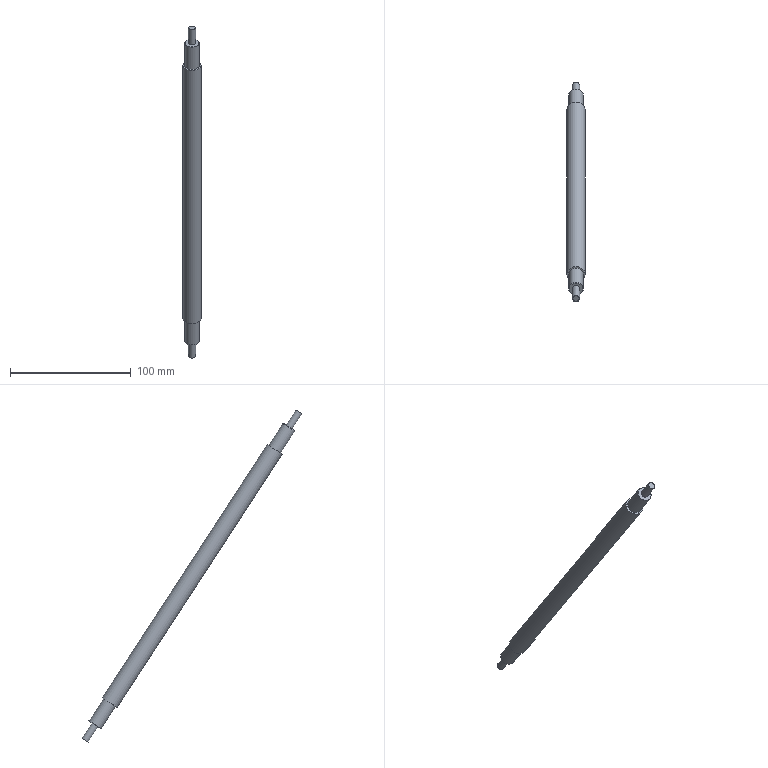Component | NX | BOTTOM_ROD | 1 solid | 13 faces | box 15 x 181.81 x 274.63 mm | volume 50002 mm3 | plane 6 | cylinder 5 | cone 2 | commonest cylinder face diameters 12 x2 6 x2 15 x1
STEP:
#1=CARTESIAN_POINT('',(0.,0.,0.));
#2=DIRECTION('',(0.,0.,1.));
#3=DIRECTION('',(1.,0.,0.));
#4=AXIS2_PLACEMENT_3D('',#1,#2,#3);
#5=CARTESIAN_POINT('',(319.193,-152.841,329.605));
#6=VERTEX_POINT('',#5);
#7=CARTESIAN_POINT('',(311.693,-152.841,329.605));
#8=DIRECTION('',(0.,-0.5459,0.8379));
#9=DIRECTION('',(1.,0.,0.));
#10=AXIS2_PLACEMENT_3D('',#7,#8,#9);
#11=CIRCLE('',#10,7.5);
#12=CARTESIAN_POINT('',(311.693,-152.841,329.605));
#13=DIRECTION('',(0.,0.5459,-0.8379));
#14=DIRECTION('',(-1.,0.,0.));
#15=AXIS2_PLACEMENT_3D('',#12,#13,#14);
#16=CYLINDRICAL_SURFACE('',#15,7.5);
#17=CARTESIAN_POINT('',(9.425,0.));
#18=DIRECTION('',(-1.,0.));
#19=VECTOR('',#18,1.);
#20=LINE('',#17,#19);
#21=(GEOMETRIC_REPRESENTATION_CONTEXT(2)PARAMETRIC_REPRESENTATION_CONTEXT()REPRESENTATION_CONTEXT('',''));
#22=DEFINITIONAL_REPRESENTATION('',(#20),#21);
#23=PCURVE('',#16,#22);
#24=CARTESIAN_POINT('',(311.693,-152.841,329.605));
#25=DIRECTION('',(0.,-0.5459,0.8379));
#26=DIRECTION('',(1.,0.,0.));
#27=AXIS2_PLACEMENT_3D('',#24,#25,#26);
#28=PLANE('',#27);
#29=CARTESIAN_POINT('',(0.,0.));
#30=DIRECTION('',(1.,0.));
#31=AXIS2_PLACEMENT_2D('',#29,#30);
#32=CIRCLE('',#31,7.5);
#33=(GEOMETRIC_REPRESENTATION_CONTEXT(2)PARAMETRIC_REPRESENTATION_CONTEXT()REPRESENTATION_CONTEXT('',''));
#34=DEFINITIONAL_REPRESENTATION('',(#32),#33);
#35=PCURVE('',#28,#34);
#36=SURFACE_CURVE('',#11,(#23,#35),.PCURVE_S1.);
#37=EDGE_CURVE('',#6,#6,#36,.T.);
#38=ORIENTED_EDGE('',*,*,#37,.F.);
#39=CARTESIAN_POINT('',(319.193,-16.376,120.136));
#40=VERTEX_POINT('',#39);
#41=CARTESIAN_POINT('',(319.193,-152.841,329.605));
#42=CARTESIAN_POINT('',(319.193,-16.376,120.136));
#43=B_SPLINE_CURVE_WITH_KNOTS('',1,(#41,#42),.UNSPECIFIED.,.F.,.F.,(2,2),(0.,250.),.PIECEWISE_BEZIER_KNOTS.);
#44=CARTESIAN_POINT('',(9.425,0.));
#45=DIRECTION('',(0.,1.));
#46=VECTOR('',#45,1.);
#47=LINE('',#44,#46);
#48=(GEOMETRIC_REPRESENTATION_CONTEXT(2)PARAMETRIC_REPRESENTATION_CONTEXT()REPRESENTATION_CONTEXT('',''));
#49=DEFINITIONAL_REPRESENTATION('',(#47),#48);
#50=PCURVE('',#16,#49);
#51=CARTESIAN_POINT('',(3.142,0.));
#52=DIRECTION('',(0.,1.));
#53=VECTOR('',#52,1.);
#54=LINE('',#51,#53);
#55=(GEOMETRIC_REPRESENTATION_CONTEXT(2)PARAMETRIC_REPRESENTATION_CONTEXT()REPRESENTATION_CONTEXT('',''));
#56=DEFINITIONAL_REPRESENTATION('',(#54),#55);
#57=PCURVE('',#16,#56);
#58=SEAM_CURVE('',#43,(#50,#57),.PCURVE_S1.);
#59=EDGE_CURVE('',#6,#40,#58,.T.);
#60=ORIENTED_EDGE('',*,*,#59,.T.);
#61=CARTESIAN_POINT('',(311.693,-16.376,120.136));
#62=DIRECTION('',(0.,-0.5459,0.8379));
#63=DIRECTION('',(1.,0.,0.));
#64=AXIS2_PLACEMENT_3D('',#61,#62,#63);
#65=CIRCLE('',#64,7.5);
#66=CARTESIAN_POINT('',(9.425,250.));
#67=DIRECTION('',(-1.,0.));
#68=VECTOR('',#67,1.);
#69=LINE('',#66,#68);
#70=(GEOMETRIC_REPRESENTATION_CONTEXT(2)PARAMETRIC_REPRESENTATION_CONTEXT()REPRESENTATION_CONTEXT('',''));
#71=DEFINITIONAL_REPRESENTATION('',(#69),#70);
#72=PCURVE('',#16,#71);
#73=CARTESIAN_POINT('',(311.693,-16.376,120.136));
#74=DIRECTION('',(0.,-0.5459,0.8379));
#75=DIRECTION('',(1.,0.,0.));
#76=AXIS2_PLACEMENT_3D('',#73,#74,#75);
#77=PLANE('',#76);
#78=CARTESIAN_POINT('',(0.,0.));
#79=DIRECTION('',(1.,0.));
#80=AXIS2_PLACEMENT_2D('',#78,#79);
#81=CIRCLE('',#80,7.5);
#82=(GEOMETRIC_REPRESENTATION_CONTEXT(2)PARAMETRIC_REPRESENTATION_CONTEXT()REPRESENTATION_CONTEXT('',''));
#83=DEFINITIONAL_REPRESENTATION('',(#81),#82);
#84=PCURVE('',#77,#83);
#85=SURFACE_CURVE('',#65,(#72,#84),.PCURVE_S1.);
#86=EDGE_CURVE('',#40,#40,#85,.T.);
#87=ORIENTED_EDGE('',*,*,#86,.T.);
#88=ORIENTED_EDGE('',*,*,#59,.F.);
#89=EDGE_LOOP('',(#38,#60,#87,#88));
#90=FACE_BOUND('',#89,.T.);
#91=ADVANCED_FACE('',(#90),#16,.T.);
#92=CARTESIAN_POINT('',(317.693,-152.841,329.605));
#93=VERTEX_POINT('',#92);
#94=CARTESIAN_POINT('',(311.693,-152.841,329.605));
#95=DIRECTION('',(0.,-0.5459,0.8379));
#96=DIRECTION('',(1.,0.,0.));
#97=AXIS2_PLACEMENT_3D('',#94,#95,#96);
#98=CIRCLE('',#97,6.);
#99=CARTESIAN_POINT('',(0.,0.));
#100=DIRECTION('',(1.,0.));
#101=AXIS2_PLACEMENT_2D('',#99,#100);
#102=CIRCLE('',#101,6.);
#103=(GEOMETRIC_REPRESENTATION_CONTEXT(2)PARAMETRIC_REPRESENTATION_CONTEXT()REPRESENTATION_CONTEXT('',''));
#104=DEFINITIONAL_REPRESENTATION('',(#102),#103);
#105=PCURVE('',#28,#104);
#106=CARTESIAN_POINT('',(311.693,-164.85,348.038));
#107=DIRECTION('',(0.,0.5459,-0.8379));
#108=DIRECTION('',(-1.,0.,0.));
#109=AXIS2_PLACEMENT_3D('',#106,#107,#108);
#110=CYLINDRICAL_SURFACE('',#109,6.);
#111=CARTESIAN_POINT('',(9.425,22.));
#112=DIRECTION('',(-1.,0.));
#113=VECTOR('',#112,1.);
#114=LINE('',#111,#113);
#115=(GEOMETRIC_REPRESENTATION_CONTEXT(2)PARAMETRIC_REPRESENTATION_CONTEXT()REPRESENTATION_CONTEXT('',''));
#116=DEFINITIONAL_REPRESENTATION('',(#114),#115);
#117=PCURVE('',#110,#116);
#118=SURFACE_CURVE('',#98,(#105,#117),.PCURVE_S1.);
#119=EDGE_CURVE('',#93,#93,#118,.T.);
#120=ORIENTED_EDGE('',*,*,#119,.F.);
#121=EDGE_LOOP('',(#120));
#122=FACE_BOUND('',#121,.T.);
#123=ORIENTED_EDGE('',*,*,#37,.T.);
#124=EDGE_LOOP('',(#123));
#125=FACE_BOUND('',#124,.T.);
#126=ADVANCED_FACE('',(#122,#125),#28,.T.);
#127=CARTESIAN_POINT('',(317.693,-16.376,120.136));
#128=VERTEX_POINT('',#127);
#129=CARTESIAN_POINT('',(311.693,-16.376,120.136));
#130=DIRECTION('',(0.,-0.5459,0.8379));
#131=DIRECTION('',(1.,0.,0.));
#132=AXIS2_PLACEMENT_3D('',#129,#130,#131);
#133=CIRCLE('',#132,6.);
#134=CARTESIAN_POINT('',(0.,0.));
#135=DIRECTION('',(1.,0.));
#136=AXIS2_PLACEMENT_2D('',#134,#135);
#137=CIRCLE('',#136,6.);
#138=(GEOMETRIC_REPRESENTATION_CONTEXT(2)PARAMETRIC_REPRESENTATION_CONTEXT()REPRESENTATION_CONTEXT('',''));
#139=DEFINITIONAL_REPRESENTATION('',(#137),#138);
#140=PCURVE('',#77,#139);
#141=CARTESIAN_POINT('',(311.693,-4.367,101.703));
#142=DIRECTION('',(0.,-0.5459,0.8379));
#143=DIRECTION('',(1.,0.,0.));
#144=AXIS2_PLACEMENT_3D('',#141,#142,#143);
#145=CYLINDRICAL_SURFACE('',#144,6.);
#146=CARTESIAN_POINT('',(0.,22.));
#147=DIRECTION('',(1.,0.));
#148=VECTOR('',#147,1.);
#149=LINE('',#146,#148);
#150=(GEOMETRIC_REPRESENTATION_CONTEXT(2)PARAMETRIC_REPRESENTATION_CONTEXT()REPRESENTATION_CONTEXT('',''));
#151=DEFINITIONAL_REPRESENTATION('',(#149),#150);
#152=PCURVE('',#145,#151);
#153=SURFACE_CURVE('',#133,(#140,#152),.PCURVE_S1.);
#154=EDGE_CURVE('',#128,#128,#153,.T.);
#155=ORIENTED_EDGE('',*,*,#154,.T.);
#156=EDGE_LOOP('',(#155));
#157=FACE_BOUND('',#156,.T.);
#158=ORIENTED_EDGE('',*,*,#86,.F.);
#159=EDGE_LOOP('',(#158));
#160=FACE_BOUND('',#159,.T.);
#161=ADVANCED_FACE('',(#157,#160),#77,.F.);
#162=CARTESIAN_POINT('',(317.693,-164.714,347.829));
#163=VERTEX_POINT('',#162);
#164=CARTESIAN_POINT('',(311.693,-164.714,347.829));
#165=DIRECTION('',(0.,0.5459,-0.8379));
#166=DIRECTION('',(1.,0.,0.));
#167=AXIS2_PLACEMENT_3D('',#164,#165,#166);
#168=CIRCLE('',#167,6.);
#169=CARTESIAN_POINT('',(3.142,0.25));
#170=DIRECTION('',(1.,0.));
#171=VECTOR('',#170,1.);
#172=LINE('',#169,#171);
#173=(GEOMETRIC_REPRESENTATION_CONTEXT(2)PARAMETRIC_REPRESENTATION_CONTEXT()REPRESENTATION_CONTEXT('',''));
#174=DEFINITIONAL_REPRESENTATION('',(#172),#173);
#175=PCURVE('',#110,#174);
#176=CARTESIAN_POINT('',(311.693,-164.85,348.038));
#177=DIRECTION('',(0.,0.5459,-0.8379));
#178=DIRECTION('',(-1.,0.,0.));
#179=AXIS2_PLACEMENT_3D('',#176,#177,#178);
#180=CONICAL_SURFACE('',#179,5.75,0.7854);
#181=CARTESIAN_POINT('',(3.142,0.25));
#182=DIRECTION('',(1.,0.));
#183=VECTOR('',#182,1.);
#184=LINE('',#181,#183);
#185=(GEOMETRIC_REPRESENTATION_CONTEXT(2)PARAMETRIC_REPRESENTATION_CONTEXT()REPRESENTATION_CONTEXT('',''));
#186=DEFINITIONAL_REPRESENTATION('',(#184),#185);
#187=PCURVE('',#180,#186);
#188=SURFACE_CURVE('',#168,(#175,#187),.PCURVE_S1.);
#189=EDGE_CURVE('',#163,#163,#188,.T.);
#190=ORIENTED_EDGE('',*,*,#189,.T.);
#191=CARTESIAN_POINT('',(317.693,-164.714,347.829));
#192=CARTESIAN_POINT('',(317.693,-152.841,329.605));
#193=B_SPLINE_CURVE_WITH_KNOTS('',1,(#191,#192),.UNSPECIFIED.,.F.,.F.,(2,2),(0.25,22.),.PIECEWISE_BEZIER_KNOTS.);
#194=CARTESIAN_POINT('',(9.425,0.));
#195=DIRECTION('',(0.,1.));
#196=VECTOR('',#195,1.);
#197=LINE('',#194,#196);
#198=(GEOMETRIC_REPRESENTATION_CONTEXT(2)PARAMETRIC_REPRESENTATION_CONTEXT()REPRESENTATION_CONTEXT('',''));
#199=DEFINITIONAL_REPRESENTATION('',(#197),#198);
#200=PCURVE('',#110,#199);
#201=CARTESIAN_POINT('',(3.142,0.));
#202=DIRECTION('',(0.,1.));
#203=VECTOR('',#202,1.);
#204=LINE('',#201,#203);
#205=(GEOMETRIC_REPRESENTATION_CONTEXT(2)PARAMETRIC_REPRESENTATION_CONTEXT()REPRESENTATION_CONTEXT('',''));
#206=DEFINITIONAL_REPRESENTATION('',(#204),#205);
#207=PCURVE('',#110,#206);
#208=SEAM_CURVE('',#193,(#200,#207),.PCURVE_S1.);
#209=EDGE_CURVE('',#163,#93,#208,.T.);
#210=ORIENTED_EDGE('',*,*,#209,.T.);
#211=ORIENTED_EDGE('',*,*,#119,.T.);
#212=ORIENTED_EDGE('',*,*,#209,.F.);
#213=EDGE_LOOP('',(#190,#210,#211,#212));
#214=FACE_BOUND('',#213,.T.);
#215=ADVANCED_FACE('',(#214),#110,.T.);
#216=CARTESIAN_POINT('',(317.443,-164.85,348.038));
#217=VERTEX_POINT('',#216);
#218=CARTESIAN_POINT('',(311.693,-164.85,348.038));
#219=DIRECTION('',(0.,-0.5459,0.8379));
#220=DIRECTION('',(1.,0.,0.));
#221=AXIS2_PLACEMENT_3D('',#218,#219,#220);
#222=CIRCLE('',#221,5.75);
#223=CARTESIAN_POINT('',(311.693,-164.85,348.038));
#224=DIRECTION('',(0.,-0.5459,0.8379));
#225=DIRECTION('',(1.,0.,0.));
#226=AXIS2_PLACEMENT_3D('',#223,#224,#225);
#227=PLANE('',#226);
#228=CARTESIAN_POINT('',(0.,0.));
#229=DIRECTION('',(1.,0.));
#230=AXIS2_PLACEMENT_2D('',#228,#229);
#231=CIRCLE('',#230,5.75);
#232=(GEOMETRIC_REPRESENTATION_CONTEXT(2)PARAMETRIC_REPRESENTATION_CONTEXT()REPRESENTATION_CONTEXT('',''));
#233=DEFINITIONAL_REPRESENTATION('',(#231),#232);
#234=PCURVE('',#227,#233);
#235=CARTESIAN_POINT('',(9.425,0.));
#236=DIRECTION('',(-1.,0.));
#237=VECTOR('',#236,1.);
#238=LINE('',#235,#237);
#239=(GEOMETRIC_REPRESENTATION_CONTEXT(2)PARAMETRIC_REPRESENTATION_CONTEXT()REPRESENTATION_CONTEXT('',''));
#240=DEFINITIONAL_REPRESENTATION('',(#238),#239);
#241=PCURVE('',#180,#240);
#242=SURFACE_CURVE('',#222,(#234,#241),.PCURVE_S1.);
#243=EDGE_CURVE('',#217,#217,#242,.T.);
#244=ORIENTED_EDGE('',*,*,#243,.T.);
#245=EDGE_LOOP('',(#244));
#246=FACE_BOUND('',#245,.T.);
#247=CARTESIAN_POINT('',(314.693,-164.85,348.038));
#248=VERTEX_POINT('',#247);
#249=CARTESIAN_POINT('',(311.693,-164.85,348.038));
#250=DIRECTION('',(0.,-0.5459,0.8379));
#251=DIRECTION('',(1.,0.,0.));
#252=AXIS2_PLACEMENT_3D('',#249,#250,#251);
#253=CIRCLE('',#252,3.);
#254=CARTESIAN_POINT('',(0.,0.));
#255=DIRECTION('',(1.,0.));
#256=AXIS2_PLACEMENT_2D('',#254,#255);
#257=CIRCLE('',#256,3.);
#258=(GEOMETRIC_REPRESENTATION_CONTEXT(2)PARAMETRIC_REPRESENTATION_CONTEXT()REPRESENTATION_CONTEXT('',''));
#259=DEFINITIONAL_REPRESENTATION('',(#257),#258);
#260=PCURVE('',#227,#259);
#261=CARTESIAN_POINT('',(311.693,-173.038,360.607));
#262=DIRECTION('',(0.,0.5459,-0.8379));
#263=DIRECTION('',(-1.,0.,0.));
#264=AXIS2_PLACEMENT_3D('',#261,#262,#263);
#265=CYLINDRICAL_SURFACE('',#264,3.);
#266=CARTESIAN_POINT('',(9.425,15.));
#267=DIRECTION('',(-1.,0.));
#268=VECTOR('',#267,1.);
#269=LINE('',#266,#268);
#270=(GEOMETRIC_REPRESENTATION_CONTEXT(2)PARAMETRIC_REPRESENTATION_CONTEXT()REPRESENTATION_CONTEXT('',''));
#271=DEFINITIONAL_REPRESENTATION('',(#269),#270);
#272=PCURVE('',#265,#271);
#273=SURFACE_CURVE('',#253,(#260,#272),.PCURVE_S1.);
#274=EDGE_CURVE('',#248,#248,#273,.T.);
#275=ORIENTED_EDGE('',*,*,#274,.F.);
#276=EDGE_LOOP('',(#275));
#277=FACE_BOUND('',#276,.T.);
#278=ADVANCED_FACE('',(#246,#277),#227,.T.);
#279=CARTESIAN_POINT('',(314.693,-172.959,360.486));
#280=VERTEX_POINT('',#279);
#281=CARTESIAN_POINT('',(311.693,-172.959,360.486));
#282=DIRECTION('',(0.,0.5459,-0.8379));
#283=DIRECTION('',(1.,0.,0.));
#284=AXIS2_PLACEMENT_3D('',#281,#282,#283);
#285=CIRCLE('',#284,3.);
#286=CARTESIAN_POINT('',(3.142,0.1443));
#287=DIRECTION('',(1.,0.));
#288=VECTOR('',#287,1.);
#289=LINE('',#286,#288);
#290=(GEOMETRIC_REPRESENTATION_CONTEXT(2)PARAMETRIC_REPRESENTATION_CONTEXT()REPRESENTATION_CONTEXT('',''));
#291=DEFINITIONAL_REPRESENTATION('',(#289),#290);
#292=PCURVE('',#265,#291);
#293=CARTESIAN_POINT('',(311.693,-173.038,360.607));
#294=DIRECTION('',(0.,0.5459,-0.8379));
#295=DIRECTION('',(-1.,0.,0.));
#296=AXIS2_PLACEMENT_3D('',#293,#294,#295);
#297=CONICAL_SURFACE('',#296,2.75,1.047);
#298=CARTESIAN_POINT('',(3.142,0.1443));
#299=DIRECTION('',(1.,0.));
#300=VECTOR('',#299,1.);
#301=LINE('',#298,#300);
#302=(GEOMETRIC_REPRESENTATION_CONTEXT(2)PARAMETRIC_REPRESENTATION_CONTEXT()REPRESENTATION_CONTEXT('',''));
#303=DEFINITIONAL_REPRESENTATION('',(#301),#302);
#304=PCURVE('',#297,#303);
#305=SURFACE_CURVE('',#285,(#292,#304),.PCURVE_S1.);
#306=EDGE_CURVE('',#280,#280,#305,.T.);
#307=ORIENTED_EDGE('',*,*,#306,.T.);
#308=CARTESIAN_POINT('',(314.693,-172.959,360.486));
#309=CARTESIAN_POINT('',(314.693,-164.85,348.038));
#310=B_SPLINE_CURVE_WITH_KNOTS('',1,(#308,#309),.UNSPECIFIED.,.F.,.F.,(2,2),(0.1443,15.),.PIECEWISE_BEZIER_KNOTS.);
#311=CARTESIAN_POINT('',(9.425,0.));
#312=DIRECTION('',(0.,1.));
#313=VECTOR('',#312,1.);
#314=LINE('',#311,#313);
#315=(GEOMETRIC_REPRESENTATION_CONTEXT(2)PARAMETRIC_REPRESENTATION_CONTEXT()REPRESENTATION_CONTEXT('',''));
#316=DEFINITIONAL_REPRESENTATION('',(#314),#315);
#317=PCURVE('',#265,#316);
#318=CARTESIAN_POINT('',(3.142,0.));
#319=DIRECTION('',(0.,1.));
#320=VECTOR('',#319,1.);
#321=LINE('',#318,#320);
#322=(GEOMETRIC_REPRESENTATION_CONTEXT(2)PARAMETRIC_REPRESENTATION_CONTEXT()REPRESENTATION_CONTEXT('',''));
#323=DEFINITIONAL_REPRESENTATION('',(#321),#322);
#324=PCURVE('',#265,#323);
#325=SEAM_CURVE('',#310,(#317,#324),.PCURVE_S1.);
#326=EDGE_CURVE('',#280,#248,#325,.T.);
#327=ORIENTED_EDGE('',*,*,#326,.T.);
#328=ORIENTED_EDGE('',*,*,#274,.T.);
#329=ORIENTED_EDGE('',*,*,#326,.F.);
#330=EDGE_LOOP('',(#307,#327,#328,#329));
#331=FACE_BOUND('',#330,.T.);
#332=ADVANCED_FACE('',(#331),#265,.T.);
#333=CARTESIAN_POINT('',(314.443,-173.038,360.607));
#334=VERTEX_POINT('',#333);
#335=CARTESIAN_POINT('',(311.693,-173.038,360.607));
#336=DIRECTION('',(0.,-0.5459,0.8379));
#337=DIRECTION('',(1.,0.,0.));
#338=AXIS2_PLACEMENT_3D('',#335,#336,#337);
#339=CIRCLE('',#338,2.75);
#340=CARTESIAN_POINT('',(311.693,-173.038,360.607));
#341=DIRECTION('',(0.,-0.5459,0.8379));
#342=DIRECTION('',(1.,0.,0.));
#343=AXIS2_PLACEMENT_3D('',#340,#341,#342);
#344=PLANE('',#343);
#345=CARTESIAN_POINT('',(0.,0.));
#346=DIRECTION('',(1.,0.));
#347=AXIS2_PLACEMENT_2D('',#345,#346);
#348=CIRCLE('',#347,2.75);
#349=(GEOMETRIC_REPRESENTATION_CONTEXT(2)PARAMETRIC_REPRESENTATION_CONTEXT()REPRESENTATION_CONTEXT('',''));
#350=DEFINITIONAL_REPRESENTATION('',(#348),#349);
#351=PCURVE('',#344,#350);
#352=CARTESIAN_POINT('',(9.425,0.));
#353=DIRECTION('',(-1.,0.));
#354=VECTOR('',#353,1.);
#355=LINE('',#352,#354);
#356=(GEOMETRIC_REPRESENTATION_CONTEXT(2)PARAMETRIC_REPRESENTATION_CONTEXT()REPRESENTATION_CONTEXT('',''));
#357=DEFINITIONAL_REPRESENTATION('',(#355),#356);
#358=PCURVE('',#297,#357);
#359=SURFACE_CURVE('',#339,(#351,#358),.PCURVE_S1.);
#360=EDGE_CURVE('',#334,#334,#359,.T.);
#361=ORIENTED_EDGE('',*,*,#360,.T.);
#362=EDGE_LOOP('',(#361));
#363=FACE_BOUND('',#362,.T.);
#364=ADVANCED_FACE('',(#363),#344,.T.);
#365=ORIENTED_EDGE('',*,*,#306,.F.);
#366=CARTESIAN_POINT('',(314.443,-173.038,360.607));
#367=CARTESIAN_POINT('',(314.693,-172.959,360.486));
#368=B_SPLINE_CURVE_WITH_KNOTS('',1,(#366,#367),.UNSPECIFIED.,.F.,.F.,(2,2),(0.,0.2887),.PIECEWISE_BEZIER_KNOTS.);
#369=CARTESIAN_POINT('',(3.142,0.));
#370=DIRECTION('',(0.,1.));
#371=VECTOR('',#370,1.);
#372=LINE('',#369,#371);
#373=(GEOMETRIC_REPRESENTATION_CONTEXT(2)PARAMETRIC_REPRESENTATION_CONTEXT()REPRESENTATION_CONTEXT('',''));
#374=DEFINITIONAL_REPRESENTATION('',(#372),#373);
#375=PCURVE('',#297,#374);
#376=CARTESIAN_POINT('',(9.425,0.));
#377=DIRECTION('',(0.,1.));
#378=VECTOR('',#377,1.);
#379=LINE('',#376,#378);
#380=(GEOMETRIC_REPRESENTATION_CONTEXT(2)PARAMETRIC_REPRESENTATION_CONTEXT()REPRESENTATION_CONTEXT('',''));
#381=DEFINITIONAL_REPRESENTATION('',(#379),#380);
#382=PCURVE('',#297,#381);
#383=SEAM_CURVE('',#368,(#375,#382),.PCURVE_S1.);
#384=EDGE_CURVE('',#334,#280,#383,.T.);
#385=ORIENTED_EDGE('',*,*,#384,.F.);
#386=ORIENTED_EDGE('',*,*,#360,.F.);
#387=ORIENTED_EDGE('',*,*,#384,.T.);
#388=EDGE_LOOP('',(#365,#385,#386,#387));
#389=FACE_BOUND('',#388,.T.);
#390=ADVANCED_FACE('',(#389),#297,.T.);
#391=ORIENTED_EDGE('',*,*,#189,.F.);
#392=CARTESIAN_POINT('',(317.443,-164.85,348.038));
#393=CARTESIAN_POINT('',(317.693,-164.714,347.829));
#394=B_SPLINE_CURVE_WITH_KNOTS('',1,(#392,#393),.UNSPECIFIED.,.F.,.F.,(2,2),(0.,0.3536),.PIECEWISE_BEZIER_KNOTS.);
#395=CARTESIAN_POINT('',(3.142,0.));
#396=DIRECTION('',(0.,1.));
#397=VECTOR('',#396,1.);
#398=LINE('',#395,#397);
#399=(GEOMETRIC_REPRESENTATION_CONTEXT(2)PARAMETRIC_REPRESENTATION_CONTEXT()REPRESENTATION_CONTEXT('',''));
#400=DEFINITIONAL_REPRESENTATION('',(#398),#399);
#401=PCURVE('',#180,#400);
#402=CARTESIAN_POINT('',(9.425,0.));
#403=DIRECTION('',(0.,1.));
#404=VECTOR('',#403,1.);
#405=LINE('',#402,#404);
#406=(GEOMETRIC_REPRESENTATION_CONTEXT(2)PARAMETRIC_REPRESENTATION_CONTEXT()REPRESENTATION_CONTEXT('',''));
#407=DEFINITIONAL_REPRESENTATION('',(#405),#406);
#408=PCURVE('',#180,#407);
#409=SEAM_CURVE('',#394,(#401,#408),.PCURVE_S1.);
#410=EDGE_CURVE('',#217,#163,#409,.T.);
#411=ORIENTED_EDGE('',*,*,#410,.F.);
#412=ORIENTED_EDGE('',*,*,#243,.F.);
#413=ORIENTED_EDGE('',*,*,#410,.T.);
#414=EDGE_LOOP('',(#391,#411,#412,#413));
#415=FACE_BOUND('',#414,.T.);
#416=ADVANCED_FACE('',(#415),#180,.T.);
#417=CARTESIAN_POINT('',(317.693,-4.367,101.703));
#418=VERTEX_POINT('',#417);
#419=CARTESIAN_POINT('',(311.693,-4.367,101.703));
#420=DIRECTION('',(0.,-0.5459,0.8379));
#421=DIRECTION('',(1.,0.,0.));
#422=AXIS2_PLACEMENT_3D('',#419,#420,#421);
#423=CIRCLE('',#422,6.);
#424=CARTESIAN_POINT('',(0.,0.));
#425=DIRECTION('',(1.,0.));
#426=VECTOR('',#425,1.);
#427=LINE('',#424,#426);
#428=(GEOMETRIC_REPRESENTATION_CONTEXT(2)PARAMETRIC_REPRESENTATION_CONTEXT()REPRESENTATION_CONTEXT('',''));
#429=DEFINITIONAL_REPRESENTATION('',(#427),#428);
#430=PCURVE('',#145,#429);
#431=CARTESIAN_POINT('',(311.693,-4.367,101.703));
#432=DIRECTION('',(0.,-0.5459,0.8379));
#433=DIRECTION('',(1.,0.,0.));
#434=AXIS2_PLACEMENT_3D('',#431,#432,#433);
#435=PLANE('',#434);
#436=CARTESIAN_POINT('',(0.,0.));
#437=DIRECTION('',(1.,0.));
#438=AXIS2_PLACEMENT_2D('',#436,#437);
#439=CIRCLE('',#438,6.);
#440=(GEOMETRIC_REPRESENTATION_CONTEXT(2)PARAMETRIC_REPRESENTATION_CONTEXT()REPRESENTATION_CONTEXT('',''));
#441=DEFINITIONAL_REPRESENTATION('',(#439),#440);
#442=PCURVE('',#435,#441);
#443=SURFACE_CURVE('',#423,(#430,#442),.PCURVE_S1.);
#444=EDGE_CURVE('',#418,#418,#443,.T.);
#445=ORIENTED_EDGE('',*,*,#444,.T.);
#446=CARTESIAN_POINT('',(317.693,-4.367,101.703));
#447=CARTESIAN_POINT('',(317.693,-16.376,120.136));
#448=B_SPLINE_CURVE_WITH_KNOTS('',1,(#446,#447),.UNSPECIFIED.,.F.,.F.,(2,2),(0.,22.),.PIECEWISE_BEZIER_KNOTS.);
#449=CARTESIAN_POINT('',(6.283,0.));
#450=DIRECTION('',(0.,1.));
#451=VECTOR('',#450,1.);
#452=LINE('',#449,#451);
#453=(GEOMETRIC_REPRESENTATION_CONTEXT(2)PARAMETRIC_REPRESENTATION_CONTEXT()REPRESENTATION_CONTEXT('',''));
#454=DEFINITIONAL_REPRESENTATION('',(#452),#453);
#455=PCURVE('',#145,#454);
#456=CARTESIAN_POINT('',(0.,0.));
#457=DIRECTION('',(0.,1.));
#458=VECTOR('',#457,1.);
#459=LINE('',#456,#458);
#460=(GEOMETRIC_REPRESENTATION_CONTEXT(2)PARAMETRIC_REPRESENTATION_CONTEXT()REPRESENTATION_CONTEXT('',''));
#461=DEFINITIONAL_REPRESENTATION('',(#459),#460);
#462=PCURVE('',#145,#461);
#463=SEAM_CURVE('',#448,(#455,#462),.PCURVE_S1.);
#464=EDGE_CURVE('',#418,#128,#463,.T.);
#465=ORIENTED_EDGE('',*,*,#464,.T.);
#466=ORIENTED_EDGE('',*,*,#154,.F.);
#467=ORIENTED_EDGE('',*,*,#464,.F.);
#468=EDGE_LOOP('',(#445,#465,#466,#467));
#469=FACE_BOUND('',#468,.T.);
#470=ADVANCED_FACE('',(#469),#145,.T.);
#471=CARTESIAN_POINT('',(314.693,-4.367,101.703));
#472=VERTEX_POINT('',#471);
#473=CARTESIAN_POINT('',(311.693,-4.367,101.703));
#474=DIRECTION('',(0.,-0.5459,0.8379));
#475=DIRECTION('',(1.,0.,0.));
#476=AXIS2_PLACEMENT_3D('',#473,#474,#475);
#477=CIRCLE('',#476,3.);
#478=CARTESIAN_POINT('',(0.,0.));
#479=DIRECTION('',(1.,0.));
#480=AXIS2_PLACEMENT_2D('',#478,#479);
#481=CIRCLE('',#480,3.);
#482=(GEOMETRIC_REPRESENTATION_CONTEXT(2)PARAMETRIC_REPRESENTATION_CONTEXT()REPRESENTATION_CONTEXT('',''));
#483=DEFINITIONAL_REPRESENTATION('',(#481),#482);
#484=PCURVE('',#435,#483);
#485=CARTESIAN_POINT('',(311.693,3.821,89.135));
#486=DIRECTION('',(0.,-0.5459,0.8379));
#487=DIRECTION('',(1.,0.,0.));
#488=AXIS2_PLACEMENT_3D('',#485,#486,#487);
#489=CYLINDRICAL_SURFACE('',#488,3.);
#490=CARTESIAN_POINT('',(0.,15.));
#491=DIRECTION('',(1.,0.));
#492=VECTOR('',#491,1.);
#493=LINE('',#490,#492);
#494=(GEOMETRIC_REPRESENTATION_CONTEXT(2)PARAMETRIC_REPRESENTATION_CONTEXT()REPRESENTATION_CONTEXT('',''));
#495=DEFINITIONAL_REPRESENTATION('',(#493),#494);
#496=PCURVE('',#489,#495);
#497=SURFACE_CURVE('',#477,(#484,#496),.PCURVE_S1.);
#498=EDGE_CURVE('',#472,#472,#497,.T.);
#499=ORIENTED_EDGE('',*,*,#498,.T.);
#500=EDGE_LOOP('',(#499));
#501=FACE_BOUND('',#500,.T.);
#502=ORIENTED_EDGE('',*,*,#444,.F.);
#503=EDGE_LOOP('',(#502));
#504=FACE_BOUND('',#503,.T.);
#505=ADVANCED_FACE('',(#501,#504),#435,.F.);
#506=CARTESIAN_POINT('',(314.693,3.821,89.135));
#507=VERTEX_POINT('',#506);
#508=CARTESIAN_POINT('',(311.693,3.821,89.135));
#509=DIRECTION('',(0.,-0.5459,0.8379));
#510=DIRECTION('',(1.,0.,0.));
#511=AXIS2_PLACEMENT_3D('',#508,#509,#510);
#512=CIRCLE('',#511,3.);
#513=CARTESIAN_POINT('',(0.,0.));
#514=DIRECTION('',(1.,0.));
#515=VECTOR('',#514,1.);
#516=LINE('',#513,#515);
#517=(GEOMETRIC_REPRESENTATION_CONTEXT(2)PARAMETRIC_REPRESENTATION_CONTEXT()REPRESENTATION_CONTEXT('',''));
#518=DEFINITIONAL_REPRESENTATION('',(#516),#517);
#519=PCURVE('',#489,#518);
#520=CARTESIAN_POINT('',(311.693,3.821,89.135));
#521=DIRECTION('',(0.,-0.5459,0.8379));
#522=DIRECTION('',(1.,0.,0.));
#523=AXIS2_PLACEMENT_3D('',#520,#521,#522);
#524=PLANE('',#523);
#525=CARTESIAN_POINT('',(0.,0.));
#526=DIRECTION('',(1.,0.));
#527=AXIS2_PLACEMENT_2D('',#525,#526);
#528=CIRCLE('',#527,3.);
#529=(GEOMETRIC_REPRESENTATION_CONTEXT(2)PARAMETRIC_REPRESENTATION_CONTEXT()REPRESENTATION_CONTEXT('',''));
#530=DEFINITIONAL_REPRESENTATION('',(#528),#529);
#531=PCURVE('',#524,#530);
#532=SURFACE_CURVE('',#512,(#519,#531),.PCURVE_S1.);
#533=EDGE_CURVE('',#507,#507,#532,.T.);
#534=ORIENTED_EDGE('',*,*,#533,.T.);
#535=CARTESIAN_POINT('',(314.693,3.821,89.135));
#536=CARTESIAN_POINT('',(314.693,-4.367,101.703));
#537=B_SPLINE_CURVE_WITH_KNOTS('',1,(#535,#536),.UNSPECIFIED.,.F.,.F.,(2,2),(0.,15.),.PIECEWISE_BEZIER_KNOTS.);
#538=CARTESIAN_POINT('',(6.283,0.));
#539=DIRECTION('',(0.,1.));
#540=VECTOR('',#539,1.);
#541=LINE('',#538,#540);
#542=(GEOMETRIC_REPRESENTATION_CONTEXT(2)PARAMETRIC_REPRESENTATION_CONTEXT()REPRESENTATION_CONTEXT('',''));
#543=DEFINITIONAL_REPRESENTATION('',(#541),#542);
#544=PCURVE('',#489,#543);
#545=CARTESIAN_POINT('',(0.,0.));
#546=DIRECTION('',(0.,1.));
#547=VECTOR('',#546,1.);
#548=LINE('',#545,#547);
#549=(GEOMETRIC_REPRESENTATION_CONTEXT(2)PARAMETRIC_REPRESENTATION_CONTEXT()REPRESENTATION_CONTEXT('',''));
#550=DEFINITIONAL_REPRESENTATION('',(#548),#549);
#551=PCURVE('',#489,#550);
#552=SEAM_CURVE('',#537,(#544,#551),.PCURVE_S1.);
#553=EDGE_CURVE('',#507,#472,#552,.T.);
#554=ORIENTED_EDGE('',*,*,#553,.T.);
#555=ORIENTED_EDGE('',*,*,#498,.F.);
#556=ORIENTED_EDGE('',*,*,#553,.F.);
#557=EDGE_LOOP('',(#534,#554,#555,#556));
#558=FACE_BOUND('',#557,.T.);
#559=ADVANCED_FACE('',(#558),#489,.T.);
#560=ORIENTED_EDGE('',*,*,#533,.F.);
#561=EDGE_LOOP('',(#560));
#562=FACE_BOUND('',#561,.T.);
#563=ADVANCED_FACE('',(#562),#524,.F.);
#564=CLOSED_SHELL('',(#91,#126,#161,#215,#278,#332,#364,#390,#416,#470,#505,#559,#563));
#565=MANIFOLD_SOLID_BREP('',#564);
#566=(LENGTH_UNIT()NAMED_UNIT(*)SI_UNIT(.MILLI.,.METRE.));
#567=UNCERTAINTY_MEASURE_WITH_UNIT(LENGTH_MEASURE(0.00001),#566,'','');
#568=(NAMED_UNIT(*)PLANE_ANGLE_UNIT()SI_UNIT($,.RADIAN.));
#569=(NAMED_UNIT(*)SI_UNIT($,.STERADIAN.)SOLID_ANGLE_UNIT());
#570=(GEOMETRIC_REPRESENTATION_CONTEXT(3)GLOBAL_UNCERTAINTY_ASSIGNED_CONTEXT((#567))GLOBAL_UNIT_ASSIGNED_CONTEXT((#566,#568,#569))REPRESENTATION_CONTEXT('',''));
#571=ADVANCED_BREP_SHAPE_REPRESENTATION('',(#4,#565),#570);